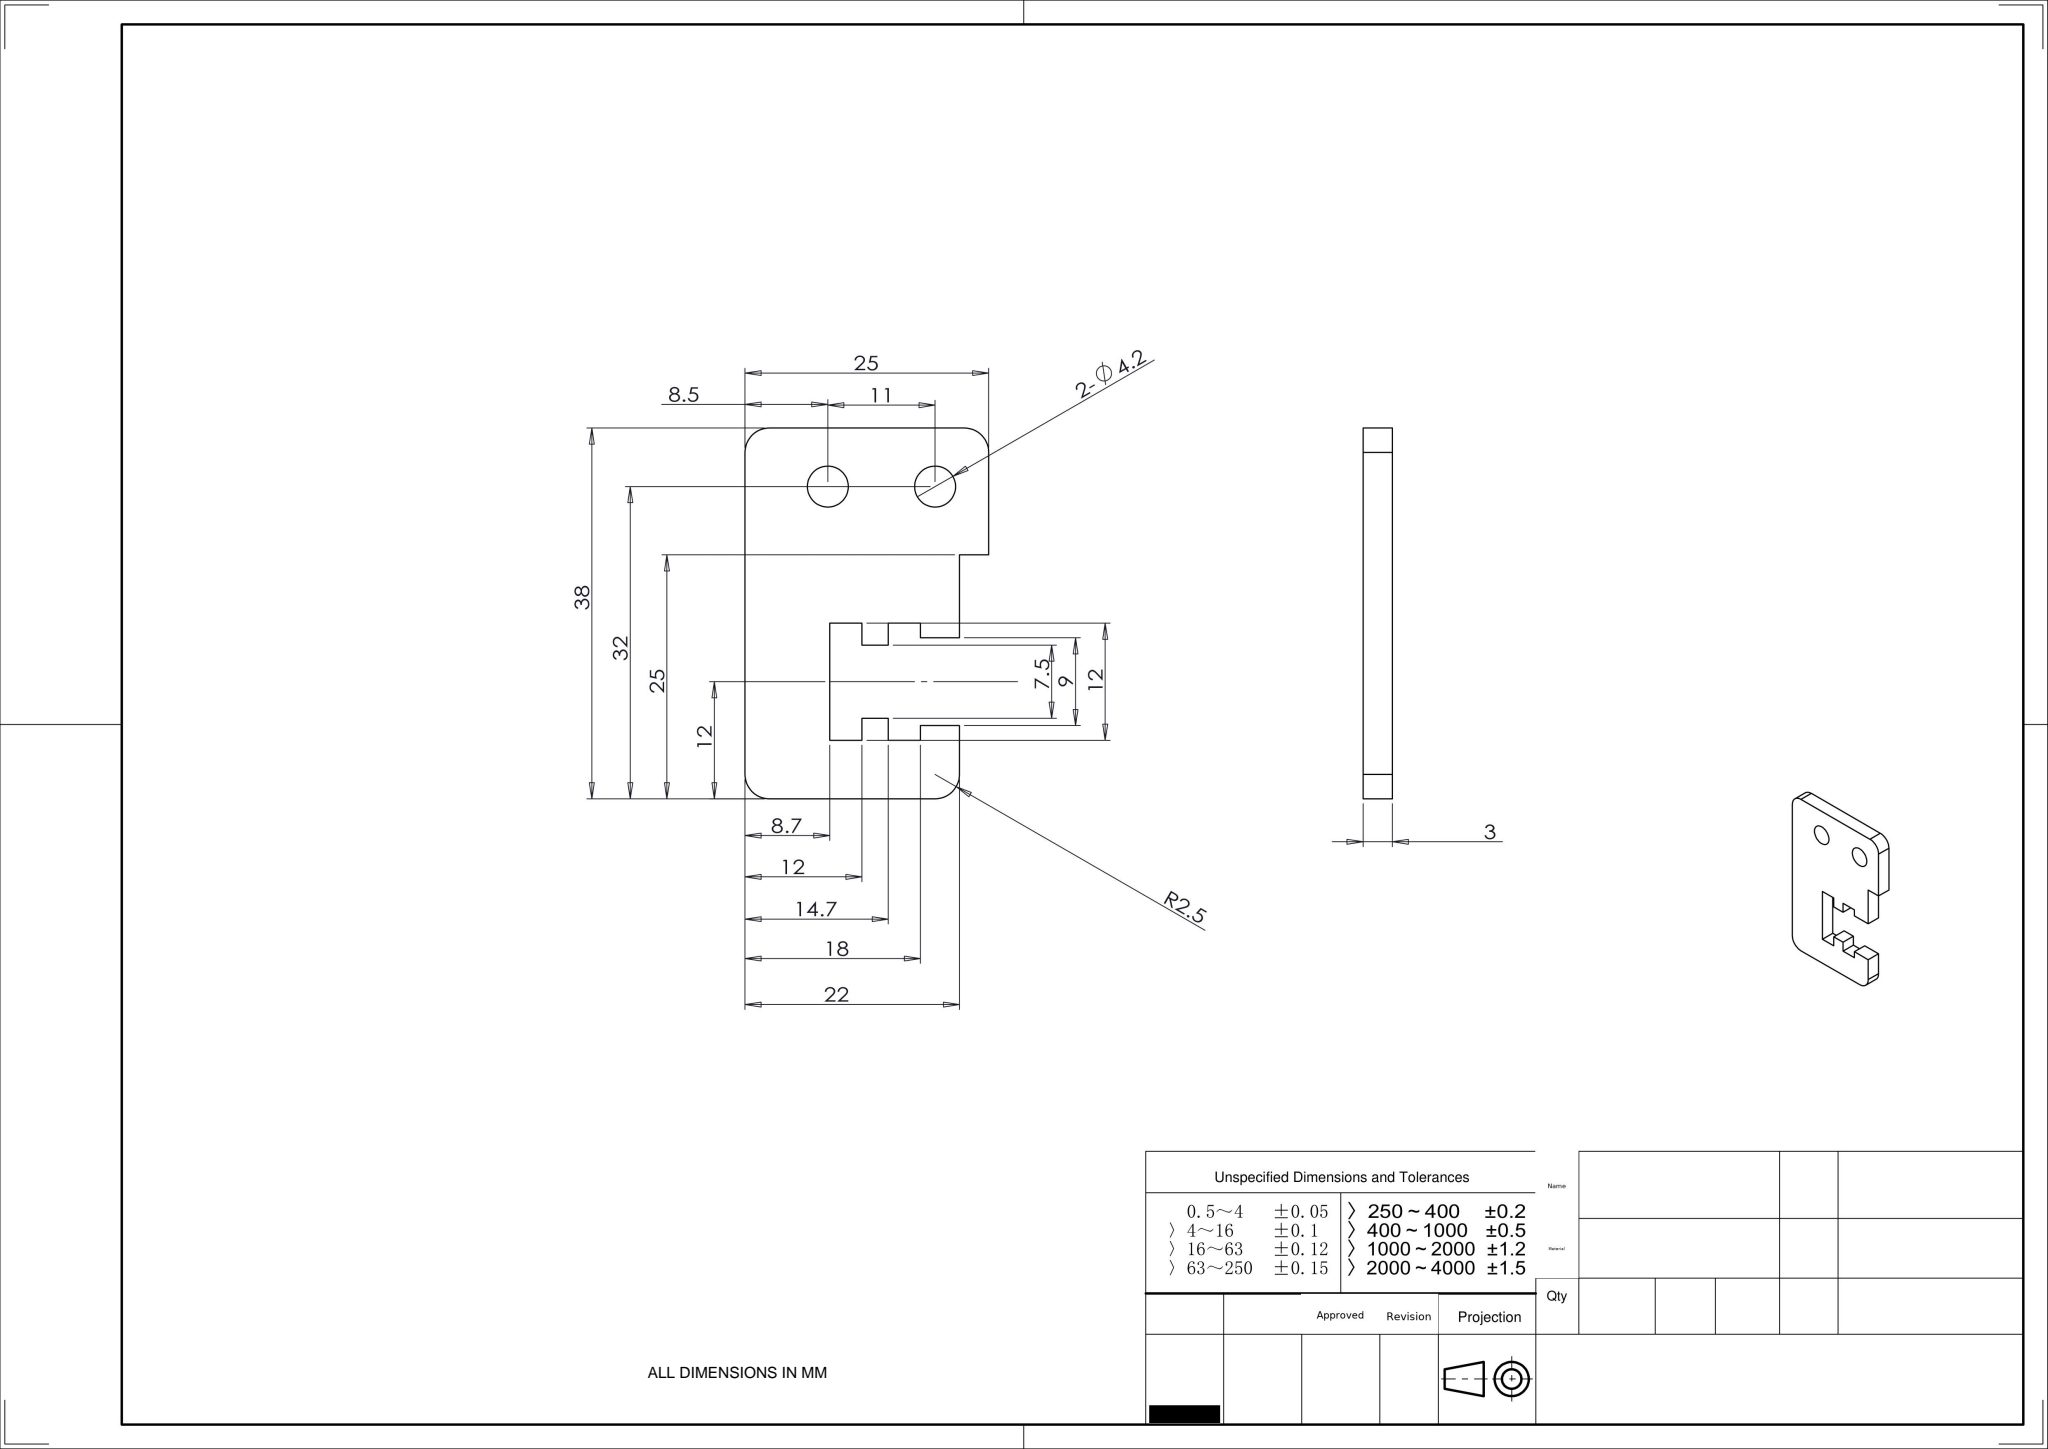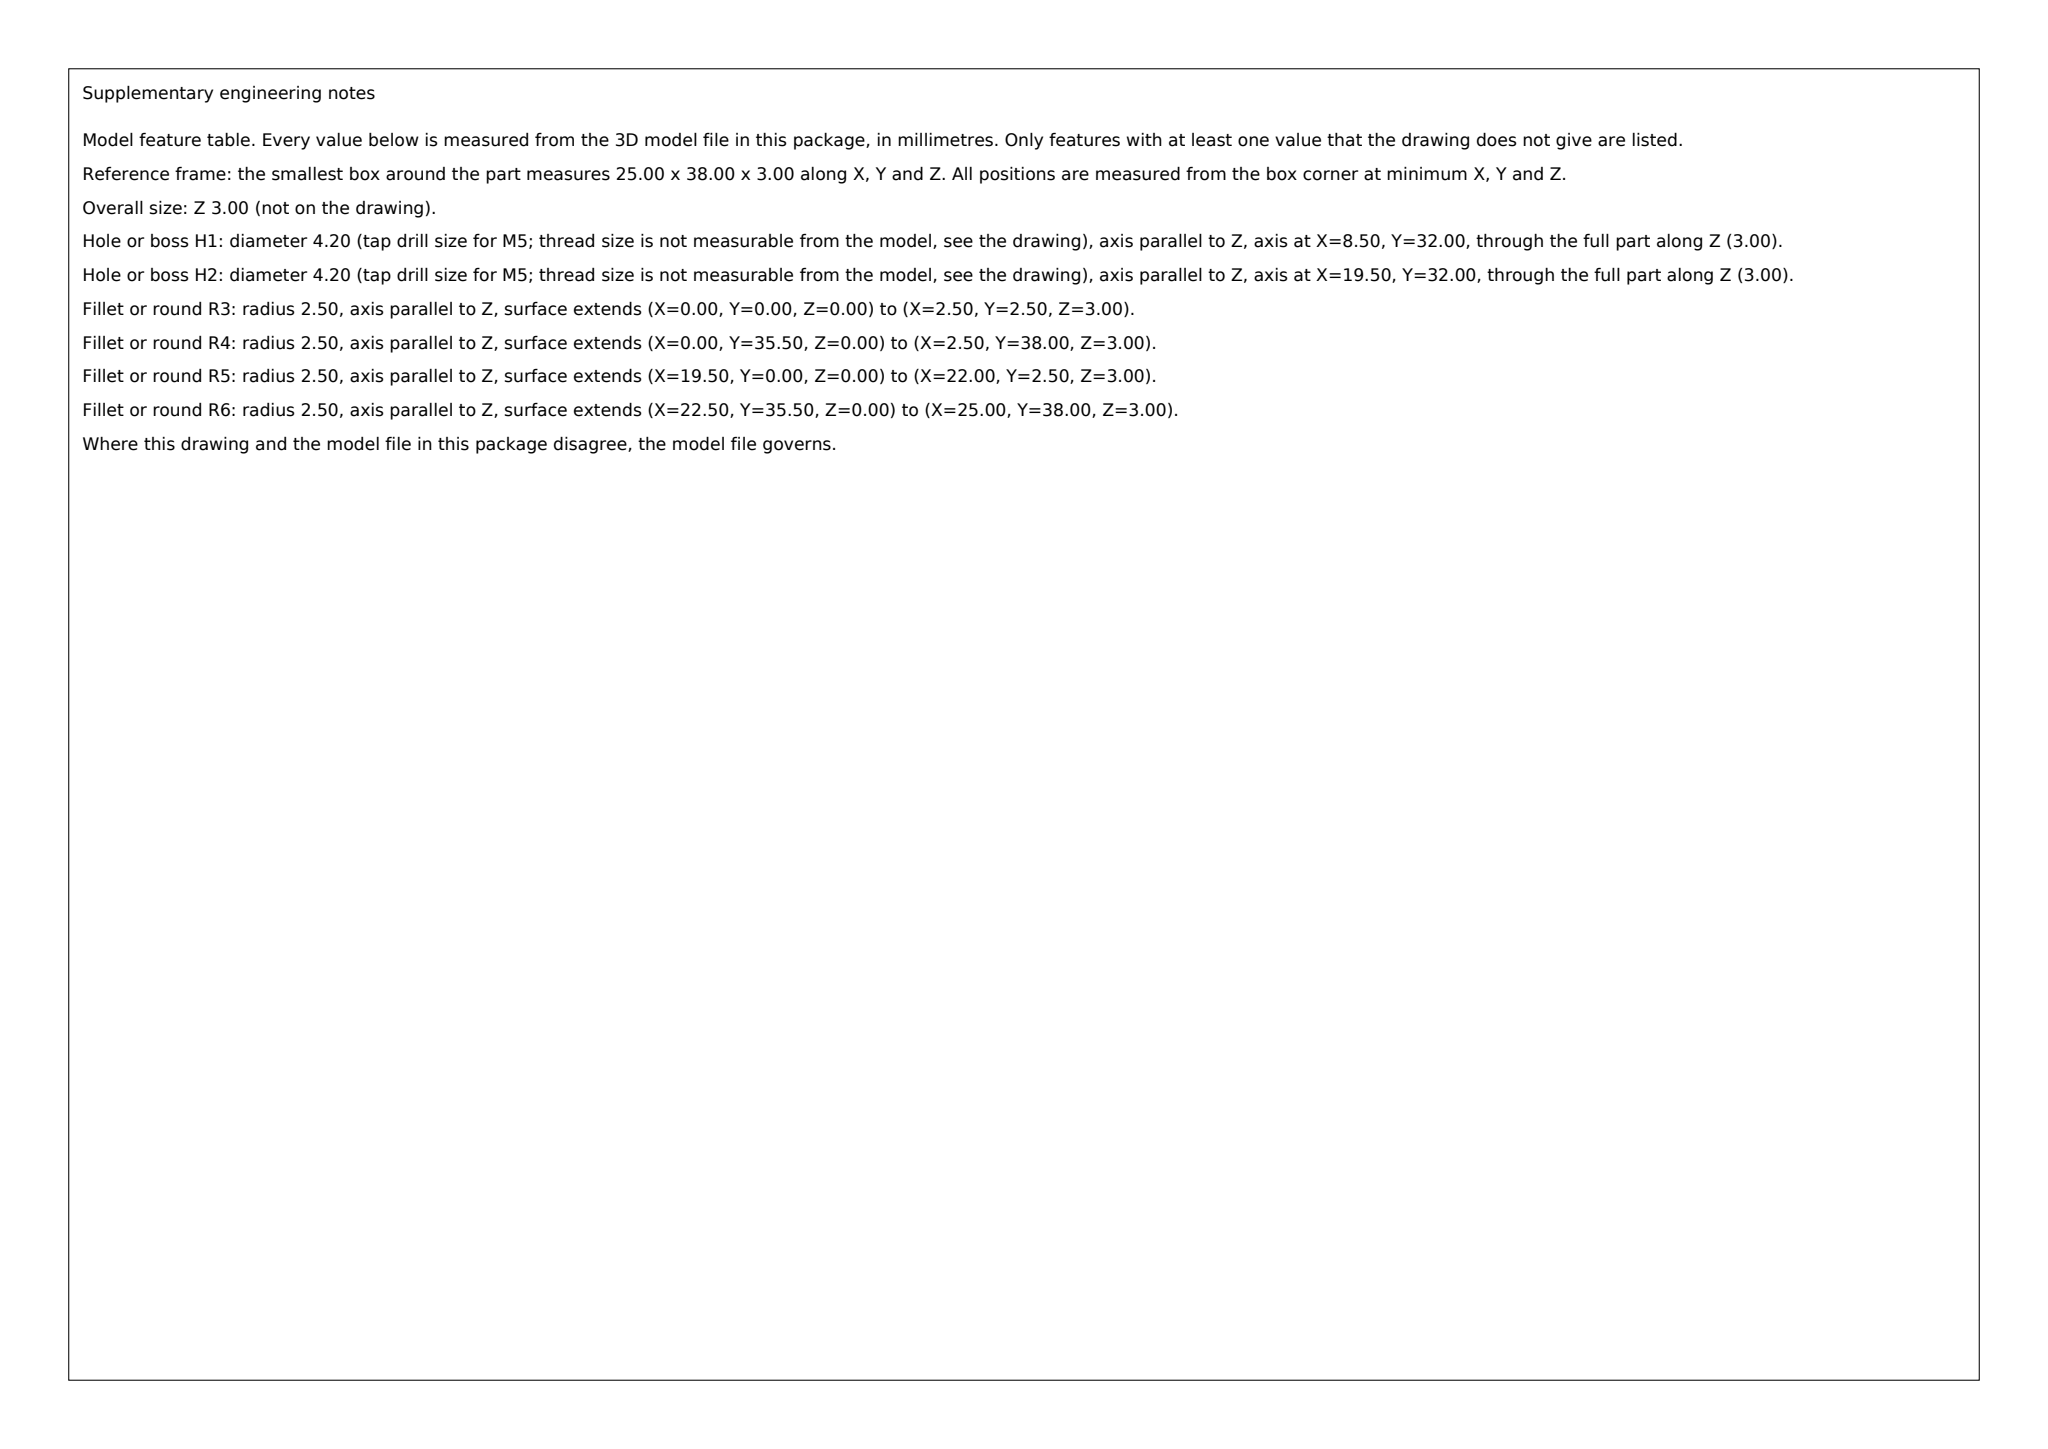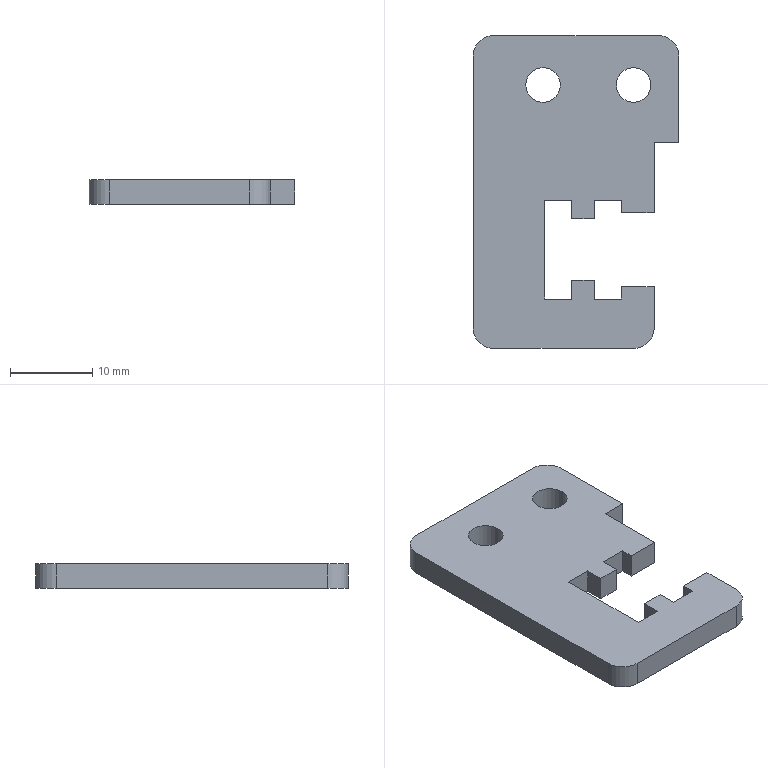Part | SolidWorks | mm | 1 solid | 32 faces | box 25 x 38 x 3 mm | volume 2119 mm3 | plane 24 | cylinder 8 | commonest cylinder face diameters 4.2 x4 5 x4